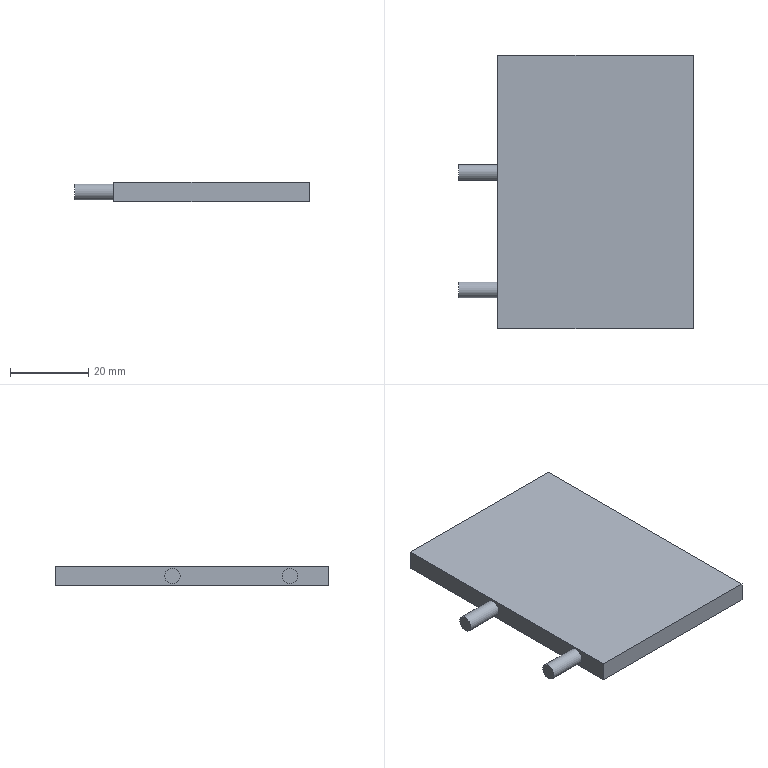Component | NX | PRINT_PLATE | 1 solid | 10 faces | box 60 x 70 x 5 mm | volume 17751 mm3 | plane 8 | cylinder 2 | commonest cylinder face diameters 4 x2
STEP:
#1=CARTESIAN_POINT('',(0.,0.,0.));
#2=DIRECTION('',(0.,0.,1.));
#3=DIRECTION('',(1.,0.,0.));
#4=AXIS2_PLACEMENT_3D('',#1,#2,#3);
#5=CARTESIAN_POINT('',(35.,110.,9.5));
#6=VERTEX_POINT('',#5);
#7=CARTESIAN_POINT('',(35.,110.,7.5));
#8=DIRECTION('',(-1.,0.,0.));
#9=DIRECTION('',(0.,0.,1.));
#10=AXIS2_PLACEMENT_3D('',#7,#8,#9);
#11=CIRCLE('',#10,2.);
#12=CARTESIAN_POINT('',(35.,140.,5.));
#13=DIRECTION('',(-1.,0.,0.));
#14=DIRECTION('',(0.,0.,1.));
#15=AXIS2_PLACEMENT_3D('',#12,#13,#14);
#16=PLANE('',#15);
#17=CARTESIAN_POINT('',(2.5,-30.));
#18=DIRECTION('',(1.,0.));
#19=AXIS2_PLACEMENT_2D('',#17,#18);
#20=CIRCLE('',#19,2.);
#21=(GEOMETRIC_REPRESENTATION_CONTEXT(2)PARAMETRIC_REPRESENTATION_CONTEXT()REPRESENTATION_CONTEXT('',''));
#22=DEFINITIONAL_REPRESENTATION('',(#20),#21);
#23=PCURVE('',#16,#22);
#24=CARTESIAN_POINT('',(25.,110.,7.5));
#25=DIRECTION('',(1.,0.,0.));
#26=DIRECTION('',(0.,0.,-1.));
#27=AXIS2_PLACEMENT_3D('',#24,#25,#26);
#28=CYLINDRICAL_SURFACE('',#27,2.);
#29=CARTESIAN_POINT('',(9.425,10.));
#30=DIRECTION('',(-1.,0.));
#31=VECTOR('',#30,1.);
#32=LINE('',#29,#31);
#33=(GEOMETRIC_REPRESENTATION_CONTEXT(2)PARAMETRIC_REPRESENTATION_CONTEXT()REPRESENTATION_CONTEXT('',''));
#34=DEFINITIONAL_REPRESENTATION('',(#32),#33);
#35=PCURVE('',#28,#34);
#36=SURFACE_CURVE('',#11,(#23,#35),.PCURVE_S1.);
#37=EDGE_CURVE('',#6,#6,#36,.T.);
#38=ORIENTED_EDGE('',*,*,#37,.F.);
#39=EDGE_LOOP('',(#38));
#40=FACE_BOUND('',#39,.T.);
#41=CARTESIAN_POINT('',(35.,80.,9.5));
#42=VERTEX_POINT('',#41);
#43=CARTESIAN_POINT('',(35.,80.,7.5));
#44=DIRECTION('',(-1.,0.,0.));
#45=DIRECTION('',(0.,0.,1.));
#46=AXIS2_PLACEMENT_3D('',#43,#44,#45);
#47=CIRCLE('',#46,2.);
#48=CARTESIAN_POINT('',(2.5,-60.));
#49=DIRECTION('',(1.,0.));
#50=AXIS2_PLACEMENT_2D('',#48,#49);
#51=CIRCLE('',#50,2.);
#52=(GEOMETRIC_REPRESENTATION_CONTEXT(2)PARAMETRIC_REPRESENTATION_CONTEXT()REPRESENTATION_CONTEXT('',''));
#53=DEFINITIONAL_REPRESENTATION('',(#51),#52);
#54=PCURVE('',#16,#53);
#55=CARTESIAN_POINT('',(25.,80.,7.5));
#56=DIRECTION('',(1.,0.,0.));
#57=DIRECTION('',(0.,0.,-1.));
#58=AXIS2_PLACEMENT_3D('',#55,#56,#57);
#59=CYLINDRICAL_SURFACE('',#58,2.);
#60=CARTESIAN_POINT('',(9.425,10.));
#61=DIRECTION('',(-1.,0.));
#62=VECTOR('',#61,1.);
#63=LINE('',#60,#62);
#64=(GEOMETRIC_REPRESENTATION_CONTEXT(2)PARAMETRIC_REPRESENTATION_CONTEXT()REPRESENTATION_CONTEXT('',''));
#65=DEFINITIONAL_REPRESENTATION('',(#63),#64);
#66=PCURVE('',#59,#65);
#67=SURFACE_CURVE('',#47,(#54,#66),.PCURVE_S1.);
#68=EDGE_CURVE('',#42,#42,#67,.T.);
#69=ORIENTED_EDGE('',*,*,#68,.F.);
#70=EDGE_LOOP('',(#69));
#71=FACE_BOUND('',#70,.T.);
#72=CARTESIAN_POINT('',(35.,140.,10.));
#73=VERTEX_POINT('',#72);
#74=CARTESIAN_POINT('',(35.,70.,10.));
#75=VERTEX_POINT('',#74);
#76=CARTESIAN_POINT('',(35.,140.,10.));
#77=DIRECTION('',(0.,-1.,0.));
#78=VECTOR('',#77,1.);
#79=LINE('',#76,#78);
#80=CARTESIAN_POINT('',(5.,0.));
#81=DIRECTION('',(0.,-1.));
#82=VECTOR('',#81,1.);
#83=LINE('',#80,#82);
#84=(GEOMETRIC_REPRESENTATION_CONTEXT(2)PARAMETRIC_REPRESENTATION_CONTEXT()REPRESENTATION_CONTEXT('',''));
#85=DEFINITIONAL_REPRESENTATION('',(#83),#84);
#86=PCURVE('',#16,#85);
#87=CARTESIAN_POINT('',(0.,0.,10.));
#88=DIRECTION('',(0.,0.,1.));
#89=DIRECTION('',(1.,0.,0.));
#90=AXIS2_PLACEMENT_3D('',#87,#88,#89);
#91=PLANE('',#90);
#92=CARTESIAN_POINT('',(35.,140.));
#93=DIRECTION('',(0.,-1.));
#94=VECTOR('',#93,1.);
#95=LINE('',#92,#94);
#96=(GEOMETRIC_REPRESENTATION_CONTEXT(2)PARAMETRIC_REPRESENTATION_CONTEXT()REPRESENTATION_CONTEXT('',''));
#97=DEFINITIONAL_REPRESENTATION('',(#95),#96);
#98=PCURVE('',#91,#97);
#99=SURFACE_CURVE('',#79,(#86,#98),.PCURVE_S1.);
#100=EDGE_CURVE('',#73,#75,#99,.T.);
#101=ORIENTED_EDGE('',*,*,#100,.F.);
#102=CARTESIAN_POINT('',(35.,140.,5.));
#103=VERTEX_POINT('',#102);
#104=CARTESIAN_POINT('',(35.,140.,5.));
#105=DIRECTION('',(0.,0.,1.));
#106=VECTOR('',#105,1.);
#107=LINE('',#104,#106);
#108=CARTESIAN_POINT('',(0.,0.));
#109=DIRECTION('',(1.,0.));
#110=VECTOR('',#109,1.);
#111=LINE('',#108,#110);
#112=(GEOMETRIC_REPRESENTATION_CONTEXT(2)PARAMETRIC_REPRESENTATION_CONTEXT()REPRESENTATION_CONTEXT('',''));
#113=DEFINITIONAL_REPRESENTATION('',(#111),#112);
#114=PCURVE('',#16,#113);
#115=CARTESIAN_POINT('',(85.,140.,5.));
#116=DIRECTION('',(0.,1.,0.));
#117=DIRECTION('',(0.,0.,1.));
#118=AXIS2_PLACEMENT_3D('',#115,#116,#117);
#119=PLANE('',#118);
#120=CARTESIAN_POINT('',(0.,-50.));
#121=DIRECTION('',(1.,0.));
#122=VECTOR('',#121,1.);
#123=LINE('',#120,#122);
#124=(GEOMETRIC_REPRESENTATION_CONTEXT(2)PARAMETRIC_REPRESENTATION_CONTEXT()REPRESENTATION_CONTEXT('',''));
#125=DEFINITIONAL_REPRESENTATION('',(#123),#124);
#126=PCURVE('',#119,#125);
#127=SURFACE_CURVE('',#107,(#114,#126),.PCURVE_S1.);
#128=EDGE_CURVE('',#103,#73,#127,.T.);
#129=ORIENTED_EDGE('',*,*,#128,.F.);
#130=CARTESIAN_POINT('',(35.,70.,5.));
#131=VERTEX_POINT('',#130);
#132=CARTESIAN_POINT('',(35.,140.,5.));
#133=DIRECTION('',(0.,-1.,0.));
#134=VECTOR('',#133,1.);
#135=LINE('',#132,#134);
#136=CARTESIAN_POINT('',(0.,0.));
#137=DIRECTION('',(0.,-1.));
#138=VECTOR('',#137,1.);
#139=LINE('',#136,#138);
#140=(GEOMETRIC_REPRESENTATION_CONTEXT(2)PARAMETRIC_REPRESENTATION_CONTEXT()REPRESENTATION_CONTEXT('',''));
#141=DEFINITIONAL_REPRESENTATION('',(#139),#140);
#142=PCURVE('',#16,#141);
#143=CARTESIAN_POINT('',(0.,0.,5.));
#144=DIRECTION('',(0.,0.,1.));
#145=DIRECTION('',(1.,0.,0.));
#146=AXIS2_PLACEMENT_3D('',#143,#144,#145);
#147=PLANE('',#146);
#148=CARTESIAN_POINT('',(35.,140.));
#149=DIRECTION('',(0.,-1.));
#150=VECTOR('',#149,1.);
#151=LINE('',#148,#150);
#152=(GEOMETRIC_REPRESENTATION_CONTEXT(2)PARAMETRIC_REPRESENTATION_CONTEXT()REPRESENTATION_CONTEXT('',''));
#153=DEFINITIONAL_REPRESENTATION('',(#151),#152);
#154=PCURVE('',#147,#153);
#155=SURFACE_CURVE('',#135,(#142,#154),.PCURVE_S1.);
#156=EDGE_CURVE('',#103,#131,#155,.T.);
#157=ORIENTED_EDGE('',*,*,#156,.T.);
#158=CARTESIAN_POINT('',(35.,70.,5.));
#159=DIRECTION('',(0.,0.,1.));
#160=VECTOR('',#159,1.);
#161=LINE('',#158,#160);
#162=CARTESIAN_POINT('',(0.,-70.));
#163=DIRECTION('',(1.,0.));
#164=VECTOR('',#163,1.);
#165=LINE('',#162,#164);
#166=(GEOMETRIC_REPRESENTATION_CONTEXT(2)PARAMETRIC_REPRESENTATION_CONTEXT()REPRESENTATION_CONTEXT('',''));
#167=DEFINITIONAL_REPRESENTATION('',(#165),#166);
#168=PCURVE('',#16,#167);
#169=CARTESIAN_POINT('',(35.,70.,5.));
#170=DIRECTION('',(0.,-1.,0.));
#171=DIRECTION('',(0.,0.,-1.));
#172=AXIS2_PLACEMENT_3D('',#169,#170,#171);
#173=PLANE('',#172);
#174=CARTESIAN_POINT('',(0.,0.));
#175=DIRECTION('',(-1.,0.));
#176=VECTOR('',#175,1.);
#177=LINE('',#174,#176);
#178=(GEOMETRIC_REPRESENTATION_CONTEXT(2)PARAMETRIC_REPRESENTATION_CONTEXT()REPRESENTATION_CONTEXT('',''));
#179=DEFINITIONAL_REPRESENTATION('',(#177),#178);
#180=PCURVE('',#173,#179);
#181=SURFACE_CURVE('',#161,(#168,#180),.PCURVE_S1.);
#182=EDGE_CURVE('',#131,#75,#181,.T.);
#183=ORIENTED_EDGE('',*,*,#182,.T.);
#184=EDGE_LOOP('',(#101,#129,#157,#183));
#185=FACE_BOUND('',#184,.T.);
#186=ADVANCED_FACE('',(#40,#71,#185),#16,.T.);
#187=CARTESIAN_POINT('',(85.,70.,10.));
#188=VERTEX_POINT('',#187);
#189=CARTESIAN_POINT('',(35.,70.,10.));
#190=DIRECTION('',(1.,0.,0.));
#191=VECTOR('',#190,1.);
#192=LINE('',#189,#191);
#193=CARTESIAN_POINT('',(-5.,0.));
#194=DIRECTION('',(0.,1.));
#195=VECTOR('',#194,1.);
#196=LINE('',#193,#195);
#197=(GEOMETRIC_REPRESENTATION_CONTEXT(2)PARAMETRIC_REPRESENTATION_CONTEXT()REPRESENTATION_CONTEXT('',''));
#198=DEFINITIONAL_REPRESENTATION('',(#196),#197);
#199=PCURVE('',#173,#198);
#200=CARTESIAN_POINT('',(35.,70.));
#201=DIRECTION('',(1.,0.));
#202=VECTOR('',#201,1.);
#203=LINE('',#200,#202);
#204=(GEOMETRIC_REPRESENTATION_CONTEXT(2)PARAMETRIC_REPRESENTATION_CONTEXT()REPRESENTATION_CONTEXT('',''));
#205=DEFINITIONAL_REPRESENTATION('',(#203),#204);
#206=PCURVE('',#91,#205);
#207=SURFACE_CURVE('',#192,(#199,#206),.PCURVE_S1.);
#208=EDGE_CURVE('',#75,#188,#207,.T.);
#209=ORIENTED_EDGE('',*,*,#208,.F.);
#210=ORIENTED_EDGE('',*,*,#182,.F.);
#211=CARTESIAN_POINT('',(85.,70.,5.));
#212=VERTEX_POINT('',#211);
#213=CARTESIAN_POINT('',(35.,70.,5.));
#214=DIRECTION('',(1.,0.,0.));
#215=VECTOR('',#214,1.);
#216=LINE('',#213,#215);
#217=CARTESIAN_POINT('',(0.,0.));
#218=DIRECTION('',(0.,1.));
#219=VECTOR('',#218,1.);
#220=LINE('',#217,#219);
#221=(GEOMETRIC_REPRESENTATION_CONTEXT(2)PARAMETRIC_REPRESENTATION_CONTEXT()REPRESENTATION_CONTEXT('',''));
#222=DEFINITIONAL_REPRESENTATION('',(#220),#221);
#223=PCURVE('',#173,#222);
#224=CARTESIAN_POINT('',(35.,70.));
#225=DIRECTION('',(1.,0.));
#226=VECTOR('',#225,1.);
#227=LINE('',#224,#226);
#228=(GEOMETRIC_REPRESENTATION_CONTEXT(2)PARAMETRIC_REPRESENTATION_CONTEXT()REPRESENTATION_CONTEXT('',''));
#229=DEFINITIONAL_REPRESENTATION('',(#227),#228);
#230=PCURVE('',#147,#229);
#231=SURFACE_CURVE('',#216,(#223,#230),.PCURVE_S1.);
#232=EDGE_CURVE('',#131,#212,#231,.T.);
#233=ORIENTED_EDGE('',*,*,#232,.T.);
#234=CARTESIAN_POINT('',(85.,70.,5.));
#235=DIRECTION('',(0.,0.,1.));
#236=VECTOR('',#235,1.);
#237=LINE('',#234,#236);
#238=CARTESIAN_POINT('',(0.,50.));
#239=DIRECTION('',(-1.,0.));
#240=VECTOR('',#239,1.);
#241=LINE('',#238,#240);
#242=(GEOMETRIC_REPRESENTATION_CONTEXT(2)PARAMETRIC_REPRESENTATION_CONTEXT()REPRESENTATION_CONTEXT('',''));
#243=DEFINITIONAL_REPRESENTATION('',(#241),#242);
#244=PCURVE('',#173,#243);
#245=CARTESIAN_POINT('',(85.,70.,5.));
#246=DIRECTION('',(1.,0.,0.));
#247=DIRECTION('',(0.,0.,-1.));
#248=AXIS2_PLACEMENT_3D('',#245,#246,#247);
#249=PLANE('',#248);
#250=CARTESIAN_POINT('',(0.,0.));
#251=DIRECTION('',(-1.,0.));
#252=VECTOR('',#251,1.);
#253=LINE('',#250,#252);
#254=(GEOMETRIC_REPRESENTATION_CONTEXT(2)PARAMETRIC_REPRESENTATION_CONTEXT()REPRESENTATION_CONTEXT('',''));
#255=DEFINITIONAL_REPRESENTATION('',(#253),#254);
#256=PCURVE('',#249,#255);
#257=SURFACE_CURVE('',#237,(#244,#256),.PCURVE_S1.);
#258=EDGE_CURVE('',#212,#188,#257,.T.);
#259=ORIENTED_EDGE('',*,*,#258,.T.);
#260=EDGE_LOOP('',(#209,#210,#233,#259));
#261=FACE_BOUND('',#260,.T.);
#262=ADVANCED_FACE('',(#261),#173,.T.);
#263=CARTESIAN_POINT('',(85.,140.,10.));
#264=VERTEX_POINT('',#263);
#265=CARTESIAN_POINT('',(85.,70.,10.));
#266=DIRECTION('',(0.,1.,0.));
#267=VECTOR('',#266,1.);
#268=LINE('',#265,#267);
#269=CARTESIAN_POINT('',(-5.,0.));
#270=DIRECTION('',(0.,1.));
#271=VECTOR('',#270,1.);
#272=LINE('',#269,#271);
#273=(GEOMETRIC_REPRESENTATION_CONTEXT(2)PARAMETRIC_REPRESENTATION_CONTEXT()REPRESENTATION_CONTEXT('',''));
#274=DEFINITIONAL_REPRESENTATION('',(#272),#273);
#275=PCURVE('',#249,#274);
#276=CARTESIAN_POINT('',(85.,70.));
#277=DIRECTION('',(0.,1.));
#278=VECTOR('',#277,1.);
#279=LINE('',#276,#278);
#280=(GEOMETRIC_REPRESENTATION_CONTEXT(2)PARAMETRIC_REPRESENTATION_CONTEXT()REPRESENTATION_CONTEXT('',''));
#281=DEFINITIONAL_REPRESENTATION('',(#279),#280);
#282=PCURVE('',#91,#281);
#283=SURFACE_CURVE('',#268,(#275,#282),.PCURVE_S1.);
#284=EDGE_CURVE('',#188,#264,#283,.T.);
#285=ORIENTED_EDGE('',*,*,#284,.F.);
#286=ORIENTED_EDGE('',*,*,#258,.F.);
#287=CARTESIAN_POINT('',(85.,140.,5.));
#288=VERTEX_POINT('',#287);
#289=CARTESIAN_POINT('',(85.,70.,5.));
#290=DIRECTION('',(0.,1.,0.));
#291=VECTOR('',#290,1.);
#292=LINE('',#289,#291);
#293=CARTESIAN_POINT('',(0.,0.));
#294=DIRECTION('',(0.,1.));
#295=VECTOR('',#294,1.);
#296=LINE('',#293,#295);
#297=(GEOMETRIC_REPRESENTATION_CONTEXT(2)PARAMETRIC_REPRESENTATION_CONTEXT()REPRESENTATION_CONTEXT('',''));
#298=DEFINITIONAL_REPRESENTATION('',(#296),#297);
#299=PCURVE('',#249,#298);
#300=CARTESIAN_POINT('',(85.,70.));
#301=DIRECTION('',(0.,1.));
#302=VECTOR('',#301,1.);
#303=LINE('',#300,#302);
#304=(GEOMETRIC_REPRESENTATION_CONTEXT(2)PARAMETRIC_REPRESENTATION_CONTEXT()REPRESENTATION_CONTEXT('',''));
#305=DEFINITIONAL_REPRESENTATION('',(#303),#304);
#306=PCURVE('',#147,#305);
#307=SURFACE_CURVE('',#292,(#299,#306),.PCURVE_S1.);
#308=EDGE_CURVE('',#212,#288,#307,.T.);
#309=ORIENTED_EDGE('',*,*,#308,.T.);
#310=CARTESIAN_POINT('',(85.,140.,5.));
#311=DIRECTION('',(0.,0.,1.));
#312=VECTOR('',#311,1.);
#313=LINE('',#310,#312);
#314=CARTESIAN_POINT('',(0.,70.));
#315=DIRECTION('',(-1.,0.));
#316=VECTOR('',#315,1.);
#317=LINE('',#314,#316);
#318=(GEOMETRIC_REPRESENTATION_CONTEXT(2)PARAMETRIC_REPRESENTATION_CONTEXT()REPRESENTATION_CONTEXT('',''));
#319=DEFINITIONAL_REPRESENTATION('',(#317),#318);
#320=PCURVE('',#249,#319);
#321=CARTESIAN_POINT('',(0.,0.));
#322=DIRECTION('',(1.,0.));
#323=VECTOR('',#322,1.);
#324=LINE('',#321,#323);
#325=(GEOMETRIC_REPRESENTATION_CONTEXT(2)PARAMETRIC_REPRESENTATION_CONTEXT()REPRESENTATION_CONTEXT('',''));
#326=DEFINITIONAL_REPRESENTATION('',(#324),#325);
#327=PCURVE('',#119,#326);
#328=SURFACE_CURVE('',#313,(#320,#327),.PCURVE_S1.);
#329=EDGE_CURVE('',#288,#264,#328,.T.);
#330=ORIENTED_EDGE('',*,*,#329,.T.);
#331=EDGE_LOOP('',(#285,#286,#309,#330));
#332=FACE_BOUND('',#331,.T.);
#333=ADVANCED_FACE('',(#332),#249,.T.);
#334=CARTESIAN_POINT('',(85.,140.,10.));
#335=DIRECTION('',(-1.,0.,0.));
#336=VECTOR('',#335,1.);
#337=LINE('',#334,#336);
#338=CARTESIAN_POINT('',(5.,0.));
#339=DIRECTION('',(0.,-1.));
#340=VECTOR('',#339,1.);
#341=LINE('',#338,#340);
#342=(GEOMETRIC_REPRESENTATION_CONTEXT(2)PARAMETRIC_REPRESENTATION_CONTEXT()REPRESENTATION_CONTEXT('',''));
#343=DEFINITIONAL_REPRESENTATION('',(#341),#342);
#344=PCURVE('',#119,#343);
#345=CARTESIAN_POINT('',(85.,140.));
#346=DIRECTION('',(-1.,0.));
#347=VECTOR('',#346,1.);
#348=LINE('',#345,#347);
#349=(GEOMETRIC_REPRESENTATION_CONTEXT(2)PARAMETRIC_REPRESENTATION_CONTEXT()REPRESENTATION_CONTEXT('',''));
#350=DEFINITIONAL_REPRESENTATION('',(#348),#349);
#351=PCURVE('',#91,#350);
#352=SURFACE_CURVE('',#337,(#344,#351),.PCURVE_S1.);
#353=EDGE_CURVE('',#264,#73,#352,.T.);
#354=ORIENTED_EDGE('',*,*,#353,.F.);
#355=ORIENTED_EDGE('',*,*,#329,.F.);
#356=CARTESIAN_POINT('',(85.,140.,5.));
#357=DIRECTION('',(-1.,0.,0.));
#358=VECTOR('',#357,1.);
#359=LINE('',#356,#358);
#360=CARTESIAN_POINT('',(0.,0.));
#361=DIRECTION('',(0.,-1.));
#362=VECTOR('',#361,1.);
#363=LINE('',#360,#362);
#364=(GEOMETRIC_REPRESENTATION_CONTEXT(2)PARAMETRIC_REPRESENTATION_CONTEXT()REPRESENTATION_CONTEXT('',''));
#365=DEFINITIONAL_REPRESENTATION('',(#363),#364);
#366=PCURVE('',#119,#365);
#367=CARTESIAN_POINT('',(85.,140.));
#368=DIRECTION('',(-1.,0.));
#369=VECTOR('',#368,1.);
#370=LINE('',#367,#369);
#371=(GEOMETRIC_REPRESENTATION_CONTEXT(2)PARAMETRIC_REPRESENTATION_CONTEXT()REPRESENTATION_CONTEXT('',''));
#372=DEFINITIONAL_REPRESENTATION('',(#370),#371);
#373=PCURVE('',#147,#372);
#374=SURFACE_CURVE('',#359,(#366,#373),.PCURVE_S1.);
#375=EDGE_CURVE('',#288,#103,#374,.T.);
#376=ORIENTED_EDGE('',*,*,#375,.T.);
#377=ORIENTED_EDGE('',*,*,#128,.T.);
#378=EDGE_LOOP('',(#354,#355,#376,#377));
#379=FACE_BOUND('',#378,.T.);
#380=ADVANCED_FACE('',(#379),#119,.T.);
#381=ORIENTED_EDGE('',*,*,#156,.F.);
#382=ORIENTED_EDGE('',*,*,#375,.F.);
#383=ORIENTED_EDGE('',*,*,#308,.F.);
#384=ORIENTED_EDGE('',*,*,#232,.F.);
#385=EDGE_LOOP('',(#381,#382,#383,#384));
#386=FACE_BOUND('',#385,.T.);
#387=ADVANCED_FACE('',(#386),#147,.F.);
#388=ORIENTED_EDGE('',*,*,#100,.T.);
#389=ORIENTED_EDGE('',*,*,#208,.T.);
#390=ORIENTED_EDGE('',*,*,#284,.T.);
#391=ORIENTED_EDGE('',*,*,#353,.T.);
#392=EDGE_LOOP('',(#388,#389,#390,#391));
#393=FACE_BOUND('',#392,.T.);
#394=ADVANCED_FACE('',(#393),#91,.T.);
#395=CARTESIAN_POINT('',(25.,80.,9.5));
#396=VERTEX_POINT('',#395);
#397=CARTESIAN_POINT('',(25.,80.,7.5));
#398=DIRECTION('',(-1.,0.,0.));
#399=DIRECTION('',(0.,0.,1.));
#400=AXIS2_PLACEMENT_3D('',#397,#398,#399);
#401=CIRCLE('',#400,2.);
#402=CARTESIAN_POINT('',(9.425,0.));
#403=DIRECTION('',(-1.,0.));
#404=VECTOR('',#403,1.);
#405=LINE('',#402,#404);
#406=(GEOMETRIC_REPRESENTATION_CONTEXT(2)PARAMETRIC_REPRESENTATION_CONTEXT()REPRESENTATION_CONTEXT('',''));
#407=DEFINITIONAL_REPRESENTATION('',(#405),#406);
#408=PCURVE('',#59,#407);
#409=CARTESIAN_POINT('',(25.,80.,7.5));
#410=DIRECTION('',(-1.,0.,0.));
#411=DIRECTION('',(0.,0.,1.));
#412=AXIS2_PLACEMENT_3D('',#409,#410,#411);
#413=PLANE('',#412);
#414=CARTESIAN_POINT('',(0.,0.));
#415=DIRECTION('',(1.,0.));
#416=AXIS2_PLACEMENT_2D('',#414,#415);
#417=CIRCLE('',#416,2.);
#418=(GEOMETRIC_REPRESENTATION_CONTEXT(2)PARAMETRIC_REPRESENTATION_CONTEXT()REPRESENTATION_CONTEXT('',''));
#419=DEFINITIONAL_REPRESENTATION('',(#417),#418);
#420=PCURVE('',#413,#419);
#421=SURFACE_CURVE('',#401,(#408,#420),.PCURVE_S1.);
#422=EDGE_CURVE('',#396,#396,#421,.T.);
#423=ORIENTED_EDGE('',*,*,#422,.F.);
#424=CARTESIAN_POINT('',(25.,80.,9.5));
#425=CARTESIAN_POINT('',(35.,80.,9.5));
#426=B_SPLINE_CURVE_WITH_KNOTS('',1,(#424,#425),.UNSPECIFIED.,.F.,.F.,(2,2),(0.,10.),.PIECEWISE_BEZIER_KNOTS.);
#427=CARTESIAN_POINT('',(9.425,0.));
#428=DIRECTION('',(0.,1.));
#429=VECTOR('',#428,1.);
#430=LINE('',#427,#429);
#431=(GEOMETRIC_REPRESENTATION_CONTEXT(2)PARAMETRIC_REPRESENTATION_CONTEXT()REPRESENTATION_CONTEXT('',''));
#432=DEFINITIONAL_REPRESENTATION('',(#430),#431);
#433=PCURVE('',#59,#432);
#434=CARTESIAN_POINT('',(3.142,0.));
#435=DIRECTION('',(0.,1.));
#436=VECTOR('',#435,1.);
#437=LINE('',#434,#436);
#438=(GEOMETRIC_REPRESENTATION_CONTEXT(2)PARAMETRIC_REPRESENTATION_CONTEXT()REPRESENTATION_CONTEXT('',''));
#439=DEFINITIONAL_REPRESENTATION('',(#437),#438);
#440=PCURVE('',#59,#439);
#441=SEAM_CURVE('',#426,(#433,#440),.PCURVE_S1.);
#442=EDGE_CURVE('',#396,#42,#441,.T.);
#443=ORIENTED_EDGE('',*,*,#442,.T.);
#444=ORIENTED_EDGE('',*,*,#68,.T.);
#445=ORIENTED_EDGE('',*,*,#442,.F.);
#446=EDGE_LOOP('',(#423,#443,#444,#445));
#447=FACE_BOUND('',#446,.T.);
#448=ADVANCED_FACE('',(#447),#59,.T.);
#449=ORIENTED_EDGE('',*,*,#422,.T.);
#450=EDGE_LOOP('',(#449));
#451=FACE_BOUND('',#450,.T.);
#452=ADVANCED_FACE('',(#451),#413,.T.);
#453=CARTESIAN_POINT('',(25.,110.,9.5));
#454=VERTEX_POINT('',#453);
#455=CARTESIAN_POINT('',(25.,110.,7.5));
#456=DIRECTION('',(-1.,0.,0.));
#457=DIRECTION('',(0.,0.,1.));
#458=AXIS2_PLACEMENT_3D('',#455,#456,#457);
#459=CIRCLE('',#458,2.);
#460=CARTESIAN_POINT('',(9.425,0.));
#461=DIRECTION('',(-1.,0.));
#462=VECTOR('',#461,1.);
#463=LINE('',#460,#462);
#464=(GEOMETRIC_REPRESENTATION_CONTEXT(2)PARAMETRIC_REPRESENTATION_CONTEXT()REPRESENTATION_CONTEXT('',''));
#465=DEFINITIONAL_REPRESENTATION('',(#463),#464);
#466=PCURVE('',#28,#465);
#467=CARTESIAN_POINT('',(25.,110.,7.5));
#468=DIRECTION('',(-1.,0.,0.));
#469=DIRECTION('',(0.,0.,1.));
#470=AXIS2_PLACEMENT_3D('',#467,#468,#469);
#471=PLANE('',#470);
#472=CARTESIAN_POINT('',(0.,0.));
#473=DIRECTION('',(1.,0.));
#474=AXIS2_PLACEMENT_2D('',#472,#473);
#475=CIRCLE('',#474,2.);
#476=(GEOMETRIC_REPRESENTATION_CONTEXT(2)PARAMETRIC_REPRESENTATION_CONTEXT()REPRESENTATION_CONTEXT('',''));
#477=DEFINITIONAL_REPRESENTATION('',(#475),#476);
#478=PCURVE('',#471,#477);
#479=SURFACE_CURVE('',#459,(#466,#478),.PCURVE_S1.);
#480=EDGE_CURVE('',#454,#454,#479,.T.);
#481=ORIENTED_EDGE('',*,*,#480,.F.);
#482=CARTESIAN_POINT('',(25.,110.,9.5));
#483=CARTESIAN_POINT('',(35.,110.,9.5));
#484=B_SPLINE_CURVE_WITH_KNOTS('',1,(#482,#483),.UNSPECIFIED.,.F.,.F.,(2,2),(0.,10.),.PIECEWISE_BEZIER_KNOTS.);
#485=CARTESIAN_POINT('',(9.425,0.));
#486=DIRECTION('',(0.,1.));
#487=VECTOR('',#486,1.);
#488=LINE('',#485,#487);
#489=(GEOMETRIC_REPRESENTATION_CONTEXT(2)PARAMETRIC_REPRESENTATION_CONTEXT()REPRESENTATION_CONTEXT('',''));
#490=DEFINITIONAL_REPRESENTATION('',(#488),#489);
#491=PCURVE('',#28,#490);
#492=CARTESIAN_POINT('',(3.142,0.));
#493=DIRECTION('',(0.,1.));
#494=VECTOR('',#493,1.);
#495=LINE('',#492,#494);
#496=(GEOMETRIC_REPRESENTATION_CONTEXT(2)PARAMETRIC_REPRESENTATION_CONTEXT()REPRESENTATION_CONTEXT('',''));
#497=DEFINITIONAL_REPRESENTATION('',(#495),#496);
#498=PCURVE('',#28,#497);
#499=SEAM_CURVE('',#484,(#491,#498),.PCURVE_S1.);
#500=EDGE_CURVE('',#454,#6,#499,.T.);
#501=ORIENTED_EDGE('',*,*,#500,.T.);
#502=ORIENTED_EDGE('',*,*,#37,.T.);
#503=ORIENTED_EDGE('',*,*,#500,.F.);
#504=EDGE_LOOP('',(#481,#501,#502,#503));
#505=FACE_BOUND('',#504,.T.);
#506=ADVANCED_FACE('',(#505),#28,.T.);
#507=ORIENTED_EDGE('',*,*,#480,.T.);
#508=EDGE_LOOP('',(#507));
#509=FACE_BOUND('',#508,.T.);
#510=ADVANCED_FACE('',(#509),#471,.T.);
#511=CLOSED_SHELL('',(#186,#262,#333,#380,#387,#394,#448,#452,#506,#510));
#512=MANIFOLD_SOLID_BREP('',#511);
#513=(LENGTH_UNIT()NAMED_UNIT(*)SI_UNIT(.MILLI.,.METRE.));
#514=UNCERTAINTY_MEASURE_WITH_UNIT(LENGTH_MEASURE(0.000002),#513,'','');
#515=(NAMED_UNIT(*)PLANE_ANGLE_UNIT()SI_UNIT($,.RADIAN.));
#516=(NAMED_UNIT(*)SI_UNIT($,.STERADIAN.)SOLID_ANGLE_UNIT());
#517=(GEOMETRIC_REPRESENTATION_CONTEXT(3)GLOBAL_UNCERTAINTY_ASSIGNED_CONTEXT((#514))GLOBAL_UNIT_ASSIGNED_CONTEXT((#513,#515,#516))REPRESENTATION_CONTEXT('',''));
#518=ADVANCED_BREP_SHAPE_REPRESENTATION('',(#4,#512),#517);